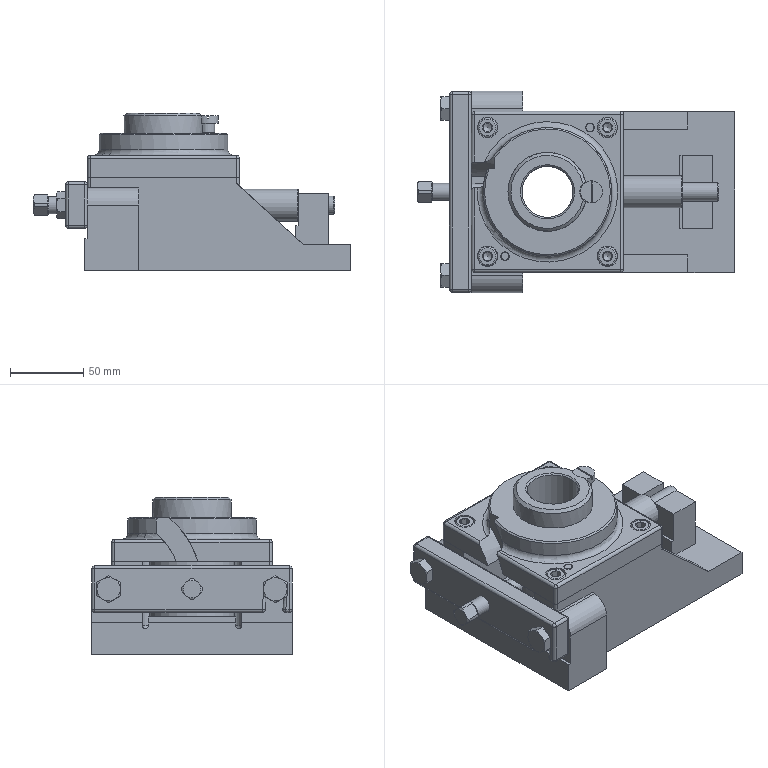Assembly | NX | mm | 15 component files | 15 solids | 407 faces | box 217 x 138 x 108 mm | volume 1120610 mm3 | plane 182 | cylinder 105 | cone 70 | torus 28 | sphere 17 | spline 5 | commonest cylinder face diameters 4 x36 6 x6 7.8 x5 7.76 x5 14.7 x4 13 x4 9 x4 14 x4
Bill of materials:
GB85-88,M12x50 | 1 |  | Square Set Screw, Long Dog Point, GB 85-88,M12x50
unnamed part 1 | 1 |  | Hollow cylindrical sleeve with a larger-diameter flange at one end. A single partial-cylinder notch cuts into the flange rim at one side. The outer edges are chamfered.
unnamed part 2 | 1 |  | Long, thin rectangular bar with rounded edges. Two round through-holes pass through the wide face. At one end, an open hook-shaped slot with a rounded inner end comes in from the bottom edge.
unnamed part 3 | 1 |  | Eye-shaped part: a short thick-walled ring with a stepped cylindrical shank sticking out sideways from its outer wall. The shank goes from a small collar at the root to a larger shaft and then a smaller-diameter end pin.
GB-T70.1-2000,M8x16 | 4 |  | Hexagon Socket Head Cap Screw, GB-T 70.1-2000,M8x16
unnamed part 4 | 1 |  | Square plate with rounded corners and a raised circular boss in the middle. A large central through-bore passes through the boss. The plate has several through-holes of different sizes, and a rectangular notch cuts in from one side edge into the boss.
GB-T119.1-2000,6x26 | 2 |  | Parallel Pin, GB-T 119.1-2000,6x26
unnamed part 5 | 1 |  | Complex prismatic block or bracket on a flat rectangular base. It has two raised side walls with a central channel between them, angled support faces, a raised pocket area with a large through-hole, small blocks on the base, and several small holes on the top faces.
GB27-88,M10x32 | 2 |  | Hex-head bolt-like part with a stepped round shank. A hexagonal head with chamfered outer edges sits on a larger shank section. A short taper leads down to a slightly smaller middle section, and a short, much smaller pilot at the end has a rounded or chamfered tip. The shank surfaces look smooth, with no threads shown.
GB830-88,M8x6 | 1 |  | Slotted Cheese Head Screw, Shoulder, GB 830-88,M8x6
Mates:
1. concentric | workpiece 1 edge | fixture_body 1 edge
2. concentric | drill_template 1 edge | fixture_body 1 arc
3. concentric | drill_bush 1 edge | drill_template 1 edge
4. concentric | clamp_plate 1 edge | fixture_body 1 arc
5. concentric | GB830-88_M8x6 1 edge | drill_bush 1 edge
6. concentric | GB27-88_M10x32 2 edge | clamp_plate 1 edge
7. concentric | GB27-88_M10x32 1 edge | clamp_plate 1 edge
8. touch align | GB85-88_M12x50 1 face | clamp_plate 1 face
9. touch align | GB85-88_M12x50 1 face | workpiece 1 face